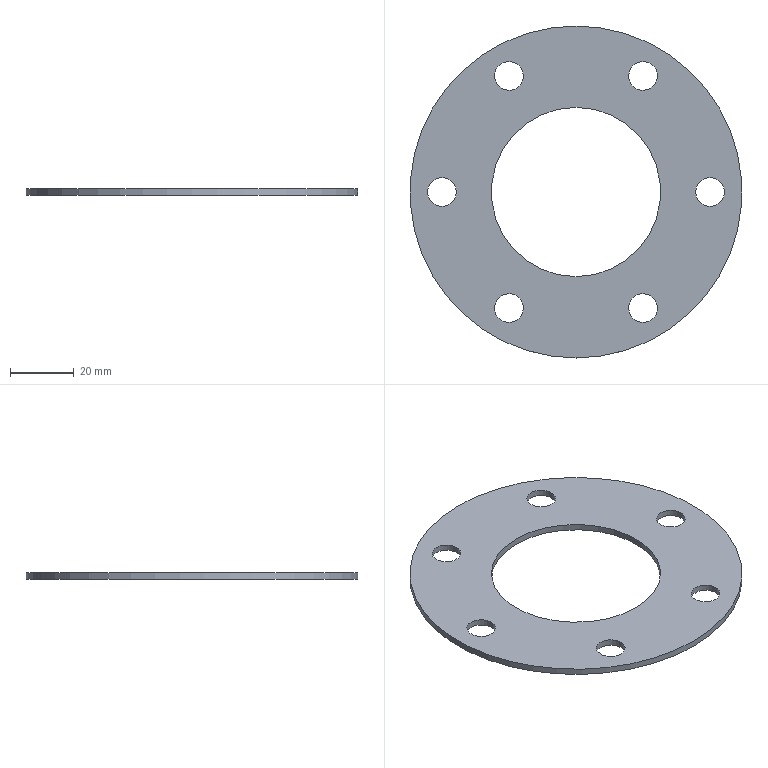Component | NX | WASHER | 1 solid | 10 faces | box 104 x 104 x 2 mm | volume 11814 mm3 | cylinder 8 | plane 2 | commonest cylinder face diameters 9 x6 53 x1 104 x1
STEP:
#1=CARTESIAN_POINT('',(0.,0.,0.));
#2=DIRECTION('',(0.,0.,1.));
#3=DIRECTION('',(1.,0.,0.));
#4=AXIS2_PLACEMENT_3D('',#1,#2,#3);
#5=CARTESIAN_POINT('',(37.397,-34.123,-67.));
#6=VERTEX_POINT('',#5);
#7=CARTESIAN_POINT('',(33.5,-36.373,-67.));
#8=DIRECTION('',(0.,0.,1.));
#9=DIRECTION('',(0.866,0.5,0.));
#10=AXIS2_PLACEMENT_3D('',#7,#8,#9);
#11=CIRCLE('',#10,4.5);
#12=CARTESIAN_POINT('',(33.5,-36.373,-67.));
#13=DIRECTION('',(0.,0.,1.));
#14=DIRECTION('',(-0.866,-0.5,0.));
#15=AXIS2_PLACEMENT_3D('',#12,#13,#14);
#16=CYLINDRICAL_SURFACE('',#15,4.5);
#17=CARTESIAN_POINT('',(3.142,0.));
#18=DIRECTION('',(1.,0.));
#19=VECTOR('',#18,1.);
#20=LINE('',#17,#19);
#21=(GEOMETRIC_REPRESENTATION_CONTEXT(2)PARAMETRIC_REPRESENTATION_CONTEXT()REPRESENTATION_CONTEXT('',''));
#22=DEFINITIONAL_REPRESENTATION('',(#20),#21);
#23=PCURVE('',#16,#22);
#24=CARTESIAN_POINT('',(23.,18.187,-67.));
#25=DIRECTION('',(0.,0.,1.));
#26=DIRECTION('',(-0.866,-0.5,0.));
#27=AXIS2_PLACEMENT_3D('',#24,#25,#26);
#28=PLANE('',#27);
#29=CARTESIAN_POINT('',(18.187,52.5));
#30=DIRECTION('',(-1.,0.));
#31=AXIS2_PLACEMENT_2D('',#29,#30);
#32=CIRCLE('',#31,4.5);
#33=(GEOMETRIC_REPRESENTATION_CONTEXT(2)PARAMETRIC_REPRESENTATION_CONTEXT()REPRESENTATION_CONTEXT('',''));
#34=DEFINITIONAL_REPRESENTATION('',(#32),#33);
#35=PCURVE('',#28,#34);
#36=SURFACE_CURVE('',#11,(#23,#35),.PCURVE_S1.);
#37=EDGE_CURVE('',#6,#6,#36,.T.);
#38=ORIENTED_EDGE('',*,*,#37,.T.);
#39=CARTESIAN_POINT('',(37.397,-34.123,-65.));
#40=VERTEX_POINT('',#39);
#41=CARTESIAN_POINT('',(37.397,-34.123,-67.));
#42=CARTESIAN_POINT('',(37.397,-34.123,-65.));
#43=B_SPLINE_CURVE_WITH_KNOTS('',1,(#41,#42),.UNSPECIFIED.,.F.,.F.,(2,2),(0.,2.),.PIECEWISE_BEZIER_KNOTS.);
#44=CARTESIAN_POINT('',(9.425,0.));
#45=DIRECTION('',(0.,1.));
#46=VECTOR('',#45,1.);
#47=LINE('',#44,#46);
#48=(GEOMETRIC_REPRESENTATION_CONTEXT(2)PARAMETRIC_REPRESENTATION_CONTEXT()REPRESENTATION_CONTEXT('',''));
#49=DEFINITIONAL_REPRESENTATION('',(#47),#48);
#50=PCURVE('',#16,#49);
#51=CARTESIAN_POINT('',(3.142,0.));
#52=DIRECTION('',(0.,1.));
#53=VECTOR('',#52,1.);
#54=LINE('',#51,#53);
#55=(GEOMETRIC_REPRESENTATION_CONTEXT(2)PARAMETRIC_REPRESENTATION_CONTEXT()REPRESENTATION_CONTEXT('',''));
#56=DEFINITIONAL_REPRESENTATION('',(#54),#55);
#57=PCURVE('',#16,#56);
#58=SEAM_CURVE('',#43,(#50,#57),.PCURVE_S1.);
#59=EDGE_CURVE('',#6,#40,#58,.T.);
#60=ORIENTED_EDGE('',*,*,#59,.T.);
#61=CARTESIAN_POINT('',(33.5,-36.373,-65.));
#62=DIRECTION('',(0.,0.,1.));
#63=DIRECTION('',(0.866,0.5,0.));
#64=AXIS2_PLACEMENT_3D('',#61,#62,#63);
#65=CIRCLE('',#64,4.5);
#66=CARTESIAN_POINT('',(3.142,2.));
#67=DIRECTION('',(1.,0.));
#68=VECTOR('',#67,1.);
#69=LINE('',#66,#68);
#70=(GEOMETRIC_REPRESENTATION_CONTEXT(2)PARAMETRIC_REPRESENTATION_CONTEXT()REPRESENTATION_CONTEXT('',''));
#71=DEFINITIONAL_REPRESENTATION('',(#69),#70);
#72=PCURVE('',#16,#71);
#73=CARTESIAN_POINT('',(23.,18.187,-65.));
#74=DIRECTION('',(0.,0.,1.));
#75=DIRECTION('',(-0.866,-0.5,0.));
#76=AXIS2_PLACEMENT_3D('',#73,#74,#75);
#77=PLANE('',#76);
#78=CARTESIAN_POINT('',(18.187,52.5));
#79=DIRECTION('',(-1.,0.));
#80=AXIS2_PLACEMENT_2D('',#78,#79);
#81=CIRCLE('',#80,4.5);
#82=(GEOMETRIC_REPRESENTATION_CONTEXT(2)PARAMETRIC_REPRESENTATION_CONTEXT()REPRESENTATION_CONTEXT('',''));
#83=DEFINITIONAL_REPRESENTATION('',(#81),#82);
#84=PCURVE('',#77,#83);
#85=SURFACE_CURVE('',#65,(#72,#84),.PCURVE_S1.);
#86=EDGE_CURVE('',#40,#40,#85,.T.);
#87=ORIENTED_EDGE('',*,*,#86,.F.);
#88=ORIENTED_EDGE('',*,*,#59,.F.);
#89=EDGE_LOOP('',(#38,#60,#87,#88));
#90=FACE_BOUND('',#89,.F.);
#91=ADVANCED_FACE('',(#90),#16,.F.);
#92=CARTESIAN_POINT('',(35.45,13.25,-67.));
#93=VERTEX_POINT('',#92);
#94=CARTESIAN_POINT('',(12.5,-0.,-67.));
#95=DIRECTION('',(0.,0.,1.));
#96=DIRECTION('',(0.866,0.5,0.));
#97=AXIS2_PLACEMENT_3D('',#94,#95,#96);
#98=CIRCLE('',#97,26.5);
#99=CARTESIAN_POINT('',(12.5,-0.,-67.));
#100=DIRECTION('',(0.,0.,1.));
#101=DIRECTION('',(-0.866,-0.5,0.));
#102=AXIS2_PLACEMENT_3D('',#99,#100,#101);
#103=CYLINDRICAL_SURFACE('',#102,26.5);
#104=CARTESIAN_POINT('',(3.142,0.));
#105=DIRECTION('',(1.,0.));
#106=VECTOR('',#105,1.);
#107=LINE('',#104,#106);
#108=(GEOMETRIC_REPRESENTATION_CONTEXT(2)PARAMETRIC_REPRESENTATION_CONTEXT()REPRESENTATION_CONTEXT('',''));
#109=DEFINITIONAL_REPRESENTATION('',(#107),#108);
#110=PCURVE('',#103,#109);
#111=CARTESIAN_POINT('',(18.187,10.5));
#112=DIRECTION('',(-1.,0.));
#113=AXIS2_PLACEMENT_2D('',#111,#112);
#114=CIRCLE('',#113,26.5);
#115=(GEOMETRIC_REPRESENTATION_CONTEXT(2)PARAMETRIC_REPRESENTATION_CONTEXT()REPRESENTATION_CONTEXT('',''));
#116=DEFINITIONAL_REPRESENTATION('',(#114),#115);
#117=PCURVE('',#28,#116);
#118=SURFACE_CURVE('',#98,(#110,#117),.PCURVE_S1.);
#119=EDGE_CURVE('',#93,#93,#118,.T.);
#120=ORIENTED_EDGE('',*,*,#119,.T.);
#121=CARTESIAN_POINT('',(35.45,13.25,-65.));
#122=VERTEX_POINT('',#121);
#123=CARTESIAN_POINT('',(35.45,13.25,-67.));
#124=CARTESIAN_POINT('',(35.45,13.25,-65.));
#125=B_SPLINE_CURVE_WITH_KNOTS('',1,(#123,#124),.UNSPECIFIED.,.F.,.F.,(2,2),(0.,2.),.PIECEWISE_BEZIER_KNOTS.);
#126=CARTESIAN_POINT('',(9.425,0.));
#127=DIRECTION('',(0.,1.));
#128=VECTOR('',#127,1.);
#129=LINE('',#126,#128);
#130=(GEOMETRIC_REPRESENTATION_CONTEXT(2)PARAMETRIC_REPRESENTATION_CONTEXT()REPRESENTATION_CONTEXT('',''));
#131=DEFINITIONAL_REPRESENTATION('',(#129),#130);
#132=PCURVE('',#103,#131);
#133=CARTESIAN_POINT('',(3.142,0.));
#134=DIRECTION('',(0.,1.));
#135=VECTOR('',#134,1.);
#136=LINE('',#133,#135);
#137=(GEOMETRIC_REPRESENTATION_CONTEXT(2)PARAMETRIC_REPRESENTATION_CONTEXT()REPRESENTATION_CONTEXT('',''));
#138=DEFINITIONAL_REPRESENTATION('',(#136),#137);
#139=PCURVE('',#103,#138);
#140=SEAM_CURVE('',#125,(#132,#139),.PCURVE_S1.);
#141=EDGE_CURVE('',#93,#122,#140,.T.);
#142=ORIENTED_EDGE('',*,*,#141,.T.);
#143=CARTESIAN_POINT('',(12.5,-0.,-65.));
#144=DIRECTION('',(0.,0.,1.));
#145=DIRECTION('',(0.866,0.5,0.));
#146=AXIS2_PLACEMENT_3D('',#143,#144,#145);
#147=CIRCLE('',#146,26.5);
#148=CARTESIAN_POINT('',(3.142,2.));
#149=DIRECTION('',(1.,0.));
#150=VECTOR('',#149,1.);
#151=LINE('',#148,#150);
#152=(GEOMETRIC_REPRESENTATION_CONTEXT(2)PARAMETRIC_REPRESENTATION_CONTEXT()REPRESENTATION_CONTEXT('',''));
#153=DEFINITIONAL_REPRESENTATION('',(#151),#152);
#154=PCURVE('',#103,#153);
#155=CARTESIAN_POINT('',(18.187,10.5));
#156=DIRECTION('',(-1.,0.));
#157=AXIS2_PLACEMENT_2D('',#155,#156);
#158=CIRCLE('',#157,26.5);
#159=(GEOMETRIC_REPRESENTATION_CONTEXT(2)PARAMETRIC_REPRESENTATION_CONTEXT()REPRESENTATION_CONTEXT('',''));
#160=DEFINITIONAL_REPRESENTATION('',(#158),#159);
#161=PCURVE('',#77,#160);
#162=SURFACE_CURVE('',#147,(#154,#161),.PCURVE_S1.);
#163=EDGE_CURVE('',#122,#122,#162,.T.);
#164=ORIENTED_EDGE('',*,*,#163,.F.);
#165=ORIENTED_EDGE('',*,*,#141,.F.);
#166=EDGE_LOOP('',(#120,#142,#164,#165));
#167=FACE_BOUND('',#166,.F.);
#168=ADVANCED_FACE('',(#167),#103,.F.);
#169=CARTESIAN_POINT('',(-29.5,-4.5,-67.));
#170=VERTEX_POINT('',#169);
#171=CARTESIAN_POINT('',(-29.5,-0.,-67.));
#172=DIRECTION('',(0.,0.,1.));
#173=DIRECTION('',(-0.,-1.,0.));
#174=AXIS2_PLACEMENT_3D('',#171,#172,#173);
#175=CIRCLE('',#174,4.5);
#176=CARTESIAN_POINT('',(-29.5,-0.,-67.));
#177=DIRECTION('',(0.,0.,1.));
#178=DIRECTION('',(-0.866,-0.5,0.));
#179=AXIS2_PLACEMENT_3D('',#176,#177,#178);
#180=CYLINDRICAL_SURFACE('',#179,4.5);
#181=CARTESIAN_POINT('',(1.047,0.));
#182=DIRECTION('',(1.,0.));
#183=VECTOR('',#182,1.);
#184=LINE('',#181,#183);
#185=(GEOMETRIC_REPRESENTATION_CONTEXT(2)PARAMETRIC_REPRESENTATION_CONTEXT()REPRESENTATION_CONTEXT('',''));
#186=DEFINITIONAL_REPRESENTATION('',(#184),#185);
#187=PCURVE('',#180,#186);
#188=CARTESIAN_POINT('',(54.56,-10.5));
#189=DIRECTION('',(0.5,0.866));
#190=AXIS2_PLACEMENT_2D('',#188,#189);
#191=CIRCLE('',#190,4.5);
#192=(GEOMETRIC_REPRESENTATION_CONTEXT(2)PARAMETRIC_REPRESENTATION_CONTEXT()REPRESENTATION_CONTEXT('',''));
#193=DEFINITIONAL_REPRESENTATION('',(#191),#192);
#194=PCURVE('',#28,#193);
#195=SURFACE_CURVE('',#175,(#187,#194),.PCURVE_S1.);
#196=EDGE_CURVE('',#170,#170,#195,.T.);
#197=ORIENTED_EDGE('',*,*,#196,.T.);
#198=CARTESIAN_POINT('',(-29.5,-4.5,-65.));
#199=VERTEX_POINT('',#198);
#200=CARTESIAN_POINT('',(-29.5,-4.5,-67.));
#201=CARTESIAN_POINT('',(-29.5,-4.5,-65.));
#202=B_SPLINE_CURVE_WITH_KNOTS('',1,(#200,#201),.UNSPECIFIED.,.F.,.F.,(2,2),(0.,2.),.PIECEWISE_BEZIER_KNOTS.);
#203=CARTESIAN_POINT('',(7.33,0.));
#204=DIRECTION('',(0.,1.));
#205=VECTOR('',#204,1.);
#206=LINE('',#203,#205);
#207=(GEOMETRIC_REPRESENTATION_CONTEXT(2)PARAMETRIC_REPRESENTATION_CONTEXT()REPRESENTATION_CONTEXT('',''));
#208=DEFINITIONAL_REPRESENTATION('',(#206),#207);
#209=PCURVE('',#180,#208);
#210=CARTESIAN_POINT('',(1.047,0.));
#211=DIRECTION('',(0.,1.));
#212=VECTOR('',#211,1.);
#213=LINE('',#210,#212);
#214=(GEOMETRIC_REPRESENTATION_CONTEXT(2)PARAMETRIC_REPRESENTATION_CONTEXT()REPRESENTATION_CONTEXT('',''));
#215=DEFINITIONAL_REPRESENTATION('',(#213),#214);
#216=PCURVE('',#180,#215);
#217=SEAM_CURVE('',#202,(#209,#216),.PCURVE_S1.);
#218=EDGE_CURVE('',#170,#199,#217,.T.);
#219=ORIENTED_EDGE('',*,*,#218,.T.);
#220=CARTESIAN_POINT('',(-29.5,-0.,-65.));
#221=DIRECTION('',(0.,0.,1.));
#222=DIRECTION('',(-0.,-1.,0.));
#223=AXIS2_PLACEMENT_3D('',#220,#221,#222);
#224=CIRCLE('',#223,4.5);
#225=CARTESIAN_POINT('',(1.047,2.));
#226=DIRECTION('',(1.,0.));
#227=VECTOR('',#226,1.);
#228=LINE('',#225,#227);
#229=(GEOMETRIC_REPRESENTATION_CONTEXT(2)PARAMETRIC_REPRESENTATION_CONTEXT()REPRESENTATION_CONTEXT('',''));
#230=DEFINITIONAL_REPRESENTATION('',(#228),#229);
#231=PCURVE('',#180,#230);
#232=CARTESIAN_POINT('',(54.56,-10.5));
#233=DIRECTION('',(0.5,0.866));
#234=AXIS2_PLACEMENT_2D('',#232,#233);
#235=CIRCLE('',#234,4.5);
#236=(GEOMETRIC_REPRESENTATION_CONTEXT(2)PARAMETRIC_REPRESENTATION_CONTEXT()REPRESENTATION_CONTEXT('',''));
#237=DEFINITIONAL_REPRESENTATION('',(#235),#236);
#238=PCURVE('',#77,#237);
#239=SURFACE_CURVE('',#224,(#231,#238),.PCURVE_S1.);
#240=EDGE_CURVE('',#199,#199,#239,.T.);
#241=ORIENTED_EDGE('',*,*,#240,.F.);
#242=ORIENTED_EDGE('',*,*,#218,.F.);
#243=EDGE_LOOP('',(#197,#219,#241,#242));
#244=FACE_BOUND('',#243,.F.);
#245=ADVANCED_FACE('',(#244),#180,.F.);
#246=CARTESIAN_POINT('',(-4.603,-38.623,-67.));
#247=VERTEX_POINT('',#246);
#248=CARTESIAN_POINT('',(-8.5,-36.373,-67.));
#249=DIRECTION('',(0.,0.,1.));
#250=DIRECTION('',(0.866,-0.5,0.));
#251=AXIS2_PLACEMENT_3D('',#248,#249,#250);
#252=CIRCLE('',#251,4.5);
#253=CARTESIAN_POINT('',(-8.5,-36.373,-67.));
#254=DIRECTION('',(0.,0.,1.));
#255=DIRECTION('',(-0.866,-0.5,0.));
#256=AXIS2_PLACEMENT_3D('',#253,#254,#255);
#257=CYLINDRICAL_SURFACE('',#256,4.5);
#258=CARTESIAN_POINT('',(2.094,0.));
#259=DIRECTION('',(1.,0.));
#260=VECTOR('',#259,1.);
#261=LINE('',#258,#260);
#262=(GEOMETRIC_REPRESENTATION_CONTEXT(2)PARAMETRIC_REPRESENTATION_CONTEXT()REPRESENTATION_CONTEXT('',''));
#263=DEFINITIONAL_REPRESENTATION('',(#261),#262);
#264=PCURVE('',#257,#263);
#265=CARTESIAN_POINT('',(54.56,31.5));
#266=DIRECTION('',(-0.5,0.866));
#267=AXIS2_PLACEMENT_2D('',#265,#266);
#268=CIRCLE('',#267,4.5);
#269=(GEOMETRIC_REPRESENTATION_CONTEXT(2)PARAMETRIC_REPRESENTATION_CONTEXT()REPRESENTATION_CONTEXT('',''));
#270=DEFINITIONAL_REPRESENTATION('',(#268),#269);
#271=PCURVE('',#28,#270);
#272=SURFACE_CURVE('',#252,(#264,#271),.PCURVE_S1.);
#273=EDGE_CURVE('',#247,#247,#272,.T.);
#274=ORIENTED_EDGE('',*,*,#273,.T.);
#275=CARTESIAN_POINT('',(-4.603,-38.623,-65.));
#276=VERTEX_POINT('',#275);
#277=CARTESIAN_POINT('',(-4.603,-38.623,-67.));
#278=CARTESIAN_POINT('',(-4.603,-38.623,-65.));
#279=B_SPLINE_CURVE_WITH_KNOTS('',1,(#277,#278),.UNSPECIFIED.,.F.,.F.,(2,2),(0.,2.),.PIECEWISE_BEZIER_KNOTS.);
#280=CARTESIAN_POINT('',(8.378,0.));
#281=DIRECTION('',(0.,1.));
#282=VECTOR('',#281,1.);
#283=LINE('',#280,#282);
#284=(GEOMETRIC_REPRESENTATION_CONTEXT(2)PARAMETRIC_REPRESENTATION_CONTEXT()REPRESENTATION_CONTEXT('',''));
#285=DEFINITIONAL_REPRESENTATION('',(#283),#284);
#286=PCURVE('',#257,#285);
#287=CARTESIAN_POINT('',(2.094,0.));
#288=DIRECTION('',(0.,1.));
#289=VECTOR('',#288,1.);
#290=LINE('',#287,#289);
#291=(GEOMETRIC_REPRESENTATION_CONTEXT(2)PARAMETRIC_REPRESENTATION_CONTEXT()REPRESENTATION_CONTEXT('',''));
#292=DEFINITIONAL_REPRESENTATION('',(#290),#291);
#293=PCURVE('',#257,#292);
#294=SEAM_CURVE('',#279,(#286,#293),.PCURVE_S1.);
#295=EDGE_CURVE('',#247,#276,#294,.T.);
#296=ORIENTED_EDGE('',*,*,#295,.T.);
#297=CARTESIAN_POINT('',(-8.5,-36.373,-65.));
#298=DIRECTION('',(0.,0.,1.));
#299=DIRECTION('',(0.866,-0.5,0.));
#300=AXIS2_PLACEMENT_3D('',#297,#298,#299);
#301=CIRCLE('',#300,4.5);
#302=CARTESIAN_POINT('',(2.094,2.));
#303=DIRECTION('',(1.,0.));
#304=VECTOR('',#303,1.);
#305=LINE('',#302,#304);
#306=(GEOMETRIC_REPRESENTATION_CONTEXT(2)PARAMETRIC_REPRESENTATION_CONTEXT()REPRESENTATION_CONTEXT('',''));
#307=DEFINITIONAL_REPRESENTATION('',(#305),#306);
#308=PCURVE('',#257,#307);
#309=CARTESIAN_POINT('',(54.56,31.5));
#310=DIRECTION('',(-0.5,0.866));
#311=AXIS2_PLACEMENT_2D('',#309,#310);
#312=CIRCLE('',#311,4.5);
#313=(GEOMETRIC_REPRESENTATION_CONTEXT(2)PARAMETRIC_REPRESENTATION_CONTEXT()REPRESENTATION_CONTEXT('',''));
#314=DEFINITIONAL_REPRESENTATION('',(#312),#313);
#315=PCURVE('',#77,#314);
#316=SURFACE_CURVE('',#301,(#308,#315),.PCURVE_S1.);
#317=EDGE_CURVE('',#276,#276,#316,.T.);
#318=ORIENTED_EDGE('',*,*,#317,.F.);
#319=ORIENTED_EDGE('',*,*,#295,.F.);
#320=EDGE_LOOP('',(#274,#296,#318,#319));
#321=FACE_BOUND('',#320,.F.);
#322=ADVANCED_FACE('',(#321),#257,.F.);
#323=CARTESIAN_POINT('',(-12.397,34.123,-67.));
#324=VERTEX_POINT('',#323);
#325=CARTESIAN_POINT('',(-8.5,36.373,-67.));
#326=DIRECTION('',(0.,0.,1.));
#327=DIRECTION('',(-0.866,-0.5,0.));
#328=AXIS2_PLACEMENT_3D('',#325,#326,#327);
#329=CIRCLE('',#328,4.5);
#330=CARTESIAN_POINT('',(-8.5,36.373,-67.));
#331=DIRECTION('',(0.,0.,1.));
#332=DIRECTION('',(-0.866,-0.5,0.));
#333=AXIS2_PLACEMENT_3D('',#330,#331,#332);
#334=CYLINDRICAL_SURFACE('',#333,4.5);
#335=CARTESIAN_POINT('',(0.,0.));
#336=DIRECTION('',(1.,0.));
#337=VECTOR('',#336,1.);
#338=LINE('',#335,#337);
#339=(GEOMETRIC_REPRESENTATION_CONTEXT(2)PARAMETRIC_REPRESENTATION_CONTEXT()REPRESENTATION_CONTEXT('',''));
#340=DEFINITIONAL_REPRESENTATION('',(#338),#339);
#341=PCURVE('',#334,#340);
#342=CARTESIAN_POINT('',(18.187,-31.5));
#343=DIRECTION('',(1.,0.));
#344=AXIS2_PLACEMENT_2D('',#342,#343);
#345=CIRCLE('',#344,4.5);
#346=(GEOMETRIC_REPRESENTATION_CONTEXT(2)PARAMETRIC_REPRESENTATION_CONTEXT()REPRESENTATION_CONTEXT('',''));
#347=DEFINITIONAL_REPRESENTATION('',(#345),#346);
#348=PCURVE('',#28,#347);
#349=SURFACE_CURVE('',#329,(#341,#348),.PCURVE_S1.);
#350=EDGE_CURVE('',#324,#324,#349,.T.);
#351=ORIENTED_EDGE('',*,*,#350,.T.);
#352=CARTESIAN_POINT('',(-12.397,34.123,-65.));
#353=VERTEX_POINT('',#352);
#354=CARTESIAN_POINT('',(-12.397,34.123,-67.));
#355=CARTESIAN_POINT('',(-12.397,34.123,-65.));
#356=B_SPLINE_CURVE_WITH_KNOTS('',1,(#354,#355),.UNSPECIFIED.,.F.,.F.,(2,2),(0.,2.),.PIECEWISE_BEZIER_KNOTS.);
#357=CARTESIAN_POINT('',(6.283,0.));
#358=DIRECTION('',(0.,1.));
#359=VECTOR('',#358,1.);
#360=LINE('',#357,#359);
#361=(GEOMETRIC_REPRESENTATION_CONTEXT(2)PARAMETRIC_REPRESENTATION_CONTEXT()REPRESENTATION_CONTEXT('',''));
#362=DEFINITIONAL_REPRESENTATION('',(#360),#361);
#363=PCURVE('',#334,#362);
#364=CARTESIAN_POINT('',(0.,0.));
#365=DIRECTION('',(0.,1.));
#366=VECTOR('',#365,1.);
#367=LINE('',#364,#366);
#368=(GEOMETRIC_REPRESENTATION_CONTEXT(2)PARAMETRIC_REPRESENTATION_CONTEXT()REPRESENTATION_CONTEXT('',''));
#369=DEFINITIONAL_REPRESENTATION('',(#367),#368);
#370=PCURVE('',#334,#369);
#371=SEAM_CURVE('',#356,(#363,#370),.PCURVE_S1.);
#372=EDGE_CURVE('',#324,#353,#371,.T.);
#373=ORIENTED_EDGE('',*,*,#372,.T.);
#374=CARTESIAN_POINT('',(-8.5,36.373,-65.));
#375=DIRECTION('',(0.,0.,1.));
#376=DIRECTION('',(-0.866,-0.5,0.));
#377=AXIS2_PLACEMENT_3D('',#374,#375,#376);
#378=CIRCLE('',#377,4.5);
#379=CARTESIAN_POINT('',(0.,2.));
#380=DIRECTION('',(1.,0.));
#381=VECTOR('',#380,1.);
#382=LINE('',#379,#381);
#383=(GEOMETRIC_REPRESENTATION_CONTEXT(2)PARAMETRIC_REPRESENTATION_CONTEXT()REPRESENTATION_CONTEXT('',''));
#384=DEFINITIONAL_REPRESENTATION('',(#382),#383);
#385=PCURVE('',#334,#384);
#386=CARTESIAN_POINT('',(18.187,-31.5));
#387=DIRECTION('',(1.,0.));
#388=AXIS2_PLACEMENT_2D('',#386,#387);
#389=CIRCLE('',#388,4.5);
#390=(GEOMETRIC_REPRESENTATION_CONTEXT(2)PARAMETRIC_REPRESENTATION_CONTEXT()REPRESENTATION_CONTEXT('',''));
#391=DEFINITIONAL_REPRESENTATION('',(#389),#390);
#392=PCURVE('',#77,#391);
#393=SURFACE_CURVE('',#378,(#385,#392),.PCURVE_S1.);
#394=EDGE_CURVE('',#353,#353,#393,.T.);
#395=ORIENTED_EDGE('',*,*,#394,.F.);
#396=ORIENTED_EDGE('',*,*,#372,.F.);
#397=EDGE_LOOP('',(#351,#373,#395,#396));
#398=FACE_BOUND('',#397,.F.);
#399=ADVANCED_FACE('',(#398),#334,.F.);
#400=CARTESIAN_POINT('',(29.603,38.623,-67.));
#401=VERTEX_POINT('',#400);
#402=CARTESIAN_POINT('',(33.5,36.373,-67.));
#403=DIRECTION('',(0.,0.,1.));
#404=DIRECTION('',(-0.866,0.5,0.));
#405=AXIS2_PLACEMENT_3D('',#402,#403,#404);
#406=CIRCLE('',#405,4.5);
#407=CARTESIAN_POINT('',(33.5,36.373,-67.));
#408=DIRECTION('',(0.,0.,1.));
#409=DIRECTION('',(-0.866,-0.5,0.));
#410=AXIS2_PLACEMENT_3D('',#407,#408,#409);
#411=CYLINDRICAL_SURFACE('',#410,4.5);
#412=CARTESIAN_POINT('',(5.236,0.));
#413=DIRECTION('',(1.,0.));
#414=VECTOR('',#413,1.);
#415=LINE('',#412,#414);
#416=(GEOMETRIC_REPRESENTATION_CONTEXT(2)PARAMETRIC_REPRESENTATION_CONTEXT()REPRESENTATION_CONTEXT('',''));
#417=DEFINITIONAL_REPRESENTATION('',(#415),#416);
#418=PCURVE('',#411,#417);
#419=CARTESIAN_POINT('',(-18.187,-10.5));
#420=DIRECTION('',(0.5,-0.866));
#421=AXIS2_PLACEMENT_2D('',#419,#420);
#422=CIRCLE('',#421,4.5);
#423=(GEOMETRIC_REPRESENTATION_CONTEXT(2)PARAMETRIC_REPRESENTATION_CONTEXT()REPRESENTATION_CONTEXT('',''));
#424=DEFINITIONAL_REPRESENTATION('',(#422),#423);
#425=PCURVE('',#28,#424);
#426=SURFACE_CURVE('',#406,(#418,#425),.PCURVE_S1.);
#427=EDGE_CURVE('',#401,#401,#426,.T.);
#428=ORIENTED_EDGE('',*,*,#427,.T.);
#429=CARTESIAN_POINT('',(29.603,38.623,-65.));
#430=VERTEX_POINT('',#429);
#431=CARTESIAN_POINT('',(29.603,38.623,-67.));
#432=CARTESIAN_POINT('',(29.603,38.623,-65.));
#433=B_SPLINE_CURVE_WITH_KNOTS('',1,(#431,#432),.UNSPECIFIED.,.F.,.F.,(2,2),(0.,2.),.PIECEWISE_BEZIER_KNOTS.);
#434=CARTESIAN_POINT('',(11.519,0.));
#435=DIRECTION('',(0.,1.));
#436=VECTOR('',#435,1.);
#437=LINE('',#434,#436);
#438=(GEOMETRIC_REPRESENTATION_CONTEXT(2)PARAMETRIC_REPRESENTATION_CONTEXT()REPRESENTATION_CONTEXT('',''));
#439=DEFINITIONAL_REPRESENTATION('',(#437),#438);
#440=PCURVE('',#411,#439);
#441=CARTESIAN_POINT('',(5.236,0.));
#442=DIRECTION('',(0.,1.));
#443=VECTOR('',#442,1.);
#444=LINE('',#441,#443);
#445=(GEOMETRIC_REPRESENTATION_CONTEXT(2)PARAMETRIC_REPRESENTATION_CONTEXT()REPRESENTATION_CONTEXT('',''));
#446=DEFINITIONAL_REPRESENTATION('',(#444),#445);
#447=PCURVE('',#411,#446);
#448=SEAM_CURVE('',#433,(#440,#447),.PCURVE_S1.);
#449=EDGE_CURVE('',#401,#430,#448,.T.);
#450=ORIENTED_EDGE('',*,*,#449,.T.);
#451=CARTESIAN_POINT('',(33.5,36.373,-65.));
#452=DIRECTION('',(0.,0.,1.));
#453=DIRECTION('',(-0.866,0.5,0.));
#454=AXIS2_PLACEMENT_3D('',#451,#452,#453);
#455=CIRCLE('',#454,4.5);
#456=CARTESIAN_POINT('',(5.236,2.));
#457=DIRECTION('',(1.,0.));
#458=VECTOR('',#457,1.);
#459=LINE('',#456,#458);
#460=(GEOMETRIC_REPRESENTATION_CONTEXT(2)PARAMETRIC_REPRESENTATION_CONTEXT()REPRESENTATION_CONTEXT('',''));
#461=DEFINITIONAL_REPRESENTATION('',(#459),#460);
#462=PCURVE('',#411,#461);
#463=CARTESIAN_POINT('',(-18.187,-10.5));
#464=DIRECTION('',(0.5,-0.866));
#465=AXIS2_PLACEMENT_2D('',#463,#464);
#466=CIRCLE('',#465,4.5);
#467=(GEOMETRIC_REPRESENTATION_CONTEXT(2)PARAMETRIC_REPRESENTATION_CONTEXT()REPRESENTATION_CONTEXT('',''));
#468=DEFINITIONAL_REPRESENTATION('',(#466),#467);
#469=PCURVE('',#77,#468);
#470=SURFACE_CURVE('',#455,(#462,#469),.PCURVE_S1.);
#471=EDGE_CURVE('',#430,#430,#470,.T.);
#472=ORIENTED_EDGE('',*,*,#471,.F.);
#473=ORIENTED_EDGE('',*,*,#449,.F.);
#474=EDGE_LOOP('',(#428,#450,#472,#473));
#475=FACE_BOUND('',#474,.F.);
#476=ADVANCED_FACE('',(#475),#411,.F.);
#477=CARTESIAN_POINT('',(57.533,26.,-67.));
#478=VERTEX_POINT('',#477);
#479=CARTESIAN_POINT('',(12.5,-0.,-67.));
#480=DIRECTION('',(0.,0.,1.));
#481=DIRECTION('',(0.866,0.5,0.));
#482=AXIS2_PLACEMENT_3D('',#479,#480,#481);
#483=CIRCLE('',#482,52.);
#484=CARTESIAN_POINT('',(12.5,-0.,-67.));
#485=DIRECTION('',(0.,0.,1.));
#486=DIRECTION('',(-0.866,-0.5,0.));
#487=AXIS2_PLACEMENT_3D('',#484,#485,#486);
#488=CYLINDRICAL_SURFACE('',#487,52.);
#489=CARTESIAN_POINT('',(3.142,0.));
#490=DIRECTION('',(1.,0.));
#491=VECTOR('',#490,1.);
#492=LINE('',#489,#491);
#493=(GEOMETRIC_REPRESENTATION_CONTEXT(2)PARAMETRIC_REPRESENTATION_CONTEXT()REPRESENTATION_CONTEXT('',''));
#494=DEFINITIONAL_REPRESENTATION('',(#492),#493);
#495=PCURVE('',#488,#494);
#496=CARTESIAN_POINT('',(18.187,10.5));
#497=DIRECTION('',(-1.,0.));
#498=AXIS2_PLACEMENT_2D('',#496,#497);
#499=CIRCLE('',#498,52.);
#500=(GEOMETRIC_REPRESENTATION_CONTEXT(2)PARAMETRIC_REPRESENTATION_CONTEXT()REPRESENTATION_CONTEXT('',''));
#501=DEFINITIONAL_REPRESENTATION('',(#499),#500);
#502=PCURVE('',#28,#501);
#503=SURFACE_CURVE('',#483,(#495,#502),.PCURVE_S1.);
#504=EDGE_CURVE('',#478,#478,#503,.T.);
#505=ORIENTED_EDGE('',*,*,#504,.T.);
#506=CARTESIAN_POINT('',(57.533,26.,-65.));
#507=VERTEX_POINT('',#506);
#508=CARTESIAN_POINT('',(57.533,26.,-67.));
#509=CARTESIAN_POINT('',(57.533,26.,-65.));
#510=B_SPLINE_CURVE_WITH_KNOTS('',1,(#508,#509),.UNSPECIFIED.,.F.,.F.,(2,2),(0.,2.),.PIECEWISE_BEZIER_KNOTS.);
#511=CARTESIAN_POINT('',(9.425,0.));
#512=DIRECTION('',(0.,1.));
#513=VECTOR('',#512,1.);
#514=LINE('',#511,#513);
#515=(GEOMETRIC_REPRESENTATION_CONTEXT(2)PARAMETRIC_REPRESENTATION_CONTEXT()REPRESENTATION_CONTEXT('',''));
#516=DEFINITIONAL_REPRESENTATION('',(#514),#515);
#517=PCURVE('',#488,#516);
#518=CARTESIAN_POINT('',(3.142,0.));
#519=DIRECTION('',(0.,1.));
#520=VECTOR('',#519,1.);
#521=LINE('',#518,#520);
#522=(GEOMETRIC_REPRESENTATION_CONTEXT(2)PARAMETRIC_REPRESENTATION_CONTEXT()REPRESENTATION_CONTEXT('',''));
#523=DEFINITIONAL_REPRESENTATION('',(#521),#522);
#524=PCURVE('',#488,#523);
#525=SEAM_CURVE('',#510,(#517,#524),.PCURVE_S1.);
#526=EDGE_CURVE('',#478,#507,#525,.T.);
#527=ORIENTED_EDGE('',*,*,#526,.T.);
#528=CARTESIAN_POINT('',(12.5,-0.,-65.));
#529=DIRECTION('',(0.,0.,1.));
#530=DIRECTION('',(0.866,0.5,0.));
#531=AXIS2_PLACEMENT_3D('',#528,#529,#530);
#532=CIRCLE('',#531,52.);
#533=CARTESIAN_POINT('',(3.142,2.));
#534=DIRECTION('',(1.,0.));
#535=VECTOR('',#534,1.);
#536=LINE('',#533,#535);
#537=(GEOMETRIC_REPRESENTATION_CONTEXT(2)PARAMETRIC_REPRESENTATION_CONTEXT()REPRESENTATION_CONTEXT('',''));
#538=DEFINITIONAL_REPRESENTATION('',(#536),#537);
#539=PCURVE('',#488,#538);
#540=CARTESIAN_POINT('',(18.187,10.5));
#541=DIRECTION('',(-1.,0.));
#542=AXIS2_PLACEMENT_2D('',#540,#541);
#543=CIRCLE('',#542,52.);
#544=(GEOMETRIC_REPRESENTATION_CONTEXT(2)PARAMETRIC_REPRESENTATION_CONTEXT()REPRESENTATION_CONTEXT('',''));
#545=DEFINITIONAL_REPRESENTATION('',(#543),#544);
#546=PCURVE('',#77,#545);
#547=SURFACE_CURVE('',#532,(#539,#546),.PCURVE_S1.);
#548=EDGE_CURVE('',#507,#507,#547,.T.);
#549=ORIENTED_EDGE('',*,*,#548,.F.);
#550=ORIENTED_EDGE('',*,*,#526,.F.);
#551=EDGE_LOOP('',(#505,#527,#549,#550));
#552=FACE_BOUND('',#551,.T.);
#553=ADVANCED_FACE('',(#552),#488,.T.);
#554=CARTESIAN_POINT('',(54.5,4.5,-67.));
#555=VERTEX_POINT('',#554);
#556=CARTESIAN_POINT('',(54.5,-0.,-67.));
#557=DIRECTION('',(0.,0.,1.));
#558=DIRECTION('',(0.,1.,0.));
#559=AXIS2_PLACEMENT_3D('',#556,#557,#558);
#560=CIRCLE('',#559,4.5);
#561=CARTESIAN_POINT('',(54.5,-0.,-67.));
#562=DIRECTION('',(0.,0.,1.));
#563=DIRECTION('',(-0.866,-0.5,0.));
#564=AXIS2_PLACEMENT_3D('',#561,#562,#563);
#565=CYLINDRICAL_SURFACE('',#564,4.5);
#566=CARTESIAN_POINT('',(4.189,0.));
#567=DIRECTION('',(1.,0.));
#568=VECTOR('',#567,1.);
#569=LINE('',#566,#568);
#570=(GEOMETRIC_REPRESENTATION_CONTEXT(2)PARAMETRIC_REPRESENTATION_CONTEXT()REPRESENTATION_CONTEXT('',''));
#571=DEFINITIONAL_REPRESENTATION('',(#569),#570);
#572=PCURVE('',#565,#571);
#573=CARTESIAN_POINT('',(-18.187,31.5));
#574=DIRECTION('',(-0.5,-0.866));
#575=AXIS2_PLACEMENT_2D('',#573,#574);
#576=CIRCLE('',#575,4.5);
#577=(GEOMETRIC_REPRESENTATION_CONTEXT(2)PARAMETRIC_REPRESENTATION_CONTEXT()REPRESENTATION_CONTEXT('',''));
#578=DEFINITIONAL_REPRESENTATION('',(#576),#577);
#579=PCURVE('',#28,#578);
#580=SURFACE_CURVE('',#560,(#572,#579),.PCURVE_S1.);
#581=EDGE_CURVE('',#555,#555,#580,.T.);
#582=ORIENTED_EDGE('',*,*,#581,.T.);
#583=CARTESIAN_POINT('',(54.5,4.5,-65.));
#584=VERTEX_POINT('',#583);
#585=CARTESIAN_POINT('',(54.5,4.5,-67.));
#586=CARTESIAN_POINT('',(54.5,4.5,-65.));
#587=B_SPLINE_CURVE_WITH_KNOTS('',1,(#585,#586),.UNSPECIFIED.,.F.,.F.,(2,2),(0.,2.),.PIECEWISE_BEZIER_KNOTS.);
#588=CARTESIAN_POINT('',(10.472,0.));
#589=DIRECTION('',(0.,1.));
#590=VECTOR('',#589,1.);
#591=LINE('',#588,#590);
#592=(GEOMETRIC_REPRESENTATION_CONTEXT(2)PARAMETRIC_REPRESENTATION_CONTEXT()REPRESENTATION_CONTEXT('',''));
#593=DEFINITIONAL_REPRESENTATION('',(#591),#592);
#594=PCURVE('',#565,#593);
#595=CARTESIAN_POINT('',(4.189,0.));
#596=DIRECTION('',(0.,1.));
#597=VECTOR('',#596,1.);
#598=LINE('',#595,#597);
#599=(GEOMETRIC_REPRESENTATION_CONTEXT(2)PARAMETRIC_REPRESENTATION_CONTEXT()REPRESENTATION_CONTEXT('',''));
#600=DEFINITIONAL_REPRESENTATION('',(#598),#599);
#601=PCURVE('',#565,#600);
#602=SEAM_CURVE('',#587,(#594,#601),.PCURVE_S1.);
#603=EDGE_CURVE('',#555,#584,#602,.T.);
#604=ORIENTED_EDGE('',*,*,#603,.T.);
#605=CARTESIAN_POINT('',(54.5,-0.,-65.));
#606=DIRECTION('',(0.,0.,1.));
#607=DIRECTION('',(0.,1.,0.));
#608=AXIS2_PLACEMENT_3D('',#605,#606,#607);
#609=CIRCLE('',#608,4.5);
#610=CARTESIAN_POINT('',(4.189,2.));
#611=DIRECTION('',(1.,0.));
#612=VECTOR('',#611,1.);
#613=LINE('',#610,#612);
#614=(GEOMETRIC_REPRESENTATION_CONTEXT(2)PARAMETRIC_REPRESENTATION_CONTEXT()REPRESENTATION_CONTEXT('',''));
#615=DEFINITIONAL_REPRESENTATION('',(#613),#614);
#616=PCURVE('',#565,#615);
#617=CARTESIAN_POINT('',(-18.187,31.5));
#618=DIRECTION('',(-0.5,-0.866));
#619=AXIS2_PLACEMENT_2D('',#617,#618);
#620=CIRCLE('',#619,4.5);
#621=(GEOMETRIC_REPRESENTATION_CONTEXT(2)PARAMETRIC_REPRESENTATION_CONTEXT()REPRESENTATION_CONTEXT('',''));
#622=DEFINITIONAL_REPRESENTATION('',(#620),#621);
#623=PCURVE('',#77,#622);
#624=SURFACE_CURVE('',#609,(#616,#623),.PCURVE_S1.);
#625=EDGE_CURVE('',#584,#584,#624,.T.);
#626=ORIENTED_EDGE('',*,*,#625,.F.);
#627=ORIENTED_EDGE('',*,*,#603,.F.);
#628=EDGE_LOOP('',(#582,#604,#626,#627));
#629=FACE_BOUND('',#628,.F.);
#630=ADVANCED_FACE('',(#629),#565,.F.);
#631=ORIENTED_EDGE('',*,*,#504,.F.);
#632=EDGE_LOOP('',(#631));
#633=FACE_BOUND('',#632,.T.);
#634=ORIENTED_EDGE('',*,*,#427,.T.);
#635=EDGE_LOOP('',(#634));
#636=FACE_BOUND('',#635,.T.);
#637=ORIENTED_EDGE('',*,*,#350,.T.);
#638=EDGE_LOOP('',(#637));
#639=FACE_BOUND('',#638,.T.);
#640=ORIENTED_EDGE('',*,*,#273,.T.);
#641=EDGE_LOOP('',(#640));
#642=FACE_BOUND('',#641,.T.);
#643=ORIENTED_EDGE('',*,*,#196,.T.);
#644=EDGE_LOOP('',(#643));
#645=FACE_BOUND('',#644,.T.);
#646=ORIENTED_EDGE('',*,*,#119,.T.);
#647=EDGE_LOOP('',(#646));
#648=FACE_BOUND('',#647,.T.);
#649=ORIENTED_EDGE('',*,*,#37,.T.);
#650=EDGE_LOOP('',(#649));
#651=FACE_BOUND('',#650,.T.);
#652=ORIENTED_EDGE('',*,*,#581,.T.);
#653=EDGE_LOOP('',(#652));
#654=FACE_BOUND('',#653,.T.);
#655=ADVANCED_FACE('',(#633,#636,#639,#642,#645,#648,#651,#654),#28,.F.);
#656=ORIENTED_EDGE('',*,*,#548,.T.);
#657=EDGE_LOOP('',(#656));
#658=FACE_BOUND('',#657,.T.);
#659=ORIENTED_EDGE('',*,*,#471,.F.);
#660=EDGE_LOOP('',(#659));
#661=FACE_BOUND('',#660,.T.);
#662=ORIENTED_EDGE('',*,*,#394,.F.);
#663=EDGE_LOOP('',(#662));
#664=FACE_BOUND('',#663,.T.);
#665=ORIENTED_EDGE('',*,*,#317,.F.);
#666=EDGE_LOOP('',(#665));
#667=FACE_BOUND('',#666,.T.);
#668=ORIENTED_EDGE('',*,*,#240,.F.);
#669=EDGE_LOOP('',(#668));
#670=FACE_BOUND('',#669,.T.);
#671=ORIENTED_EDGE('',*,*,#163,.F.);
#672=EDGE_LOOP('',(#671));
#673=FACE_BOUND('',#672,.T.);
#674=ORIENTED_EDGE('',*,*,#86,.F.);
#675=EDGE_LOOP('',(#674));
#676=FACE_BOUND('',#675,.T.);
#677=ORIENTED_EDGE('',*,*,#625,.F.);
#678=EDGE_LOOP('',(#677));
#679=FACE_BOUND('',#678,.T.);
#680=ADVANCED_FACE('',(#658,#661,#664,#667,#670,#673,#676,#679),#77,.T.);
#681=CLOSED_SHELL('',(#91,#168,#245,#322,#399,#476,#553,#630,#655,#680));
#682=MANIFOLD_SOLID_BREP('',#681);
#683=(LENGTH_UNIT()NAMED_UNIT(*)SI_UNIT(.MILLI.,.METRE.));
#684=UNCERTAINTY_MEASURE_WITH_UNIT(LENGTH_MEASURE(0.00001),#683,'','');
#685=(NAMED_UNIT(*)PLANE_ANGLE_UNIT()SI_UNIT($,.RADIAN.));
#686=(NAMED_UNIT(*)SI_UNIT($,.STERADIAN.)SOLID_ANGLE_UNIT());
#687=(GEOMETRIC_REPRESENTATION_CONTEXT(3)GLOBAL_UNCERTAINTY_ASSIGNED_CONTEXT((#684))GLOBAL_UNIT_ASSIGNED_CONTEXT((#683,#685,#686))REPRESENTATION_CONTEXT('',''));
#688=ADVANCED_BREP_SHAPE_REPRESENTATION('',(#4,#682),#687);